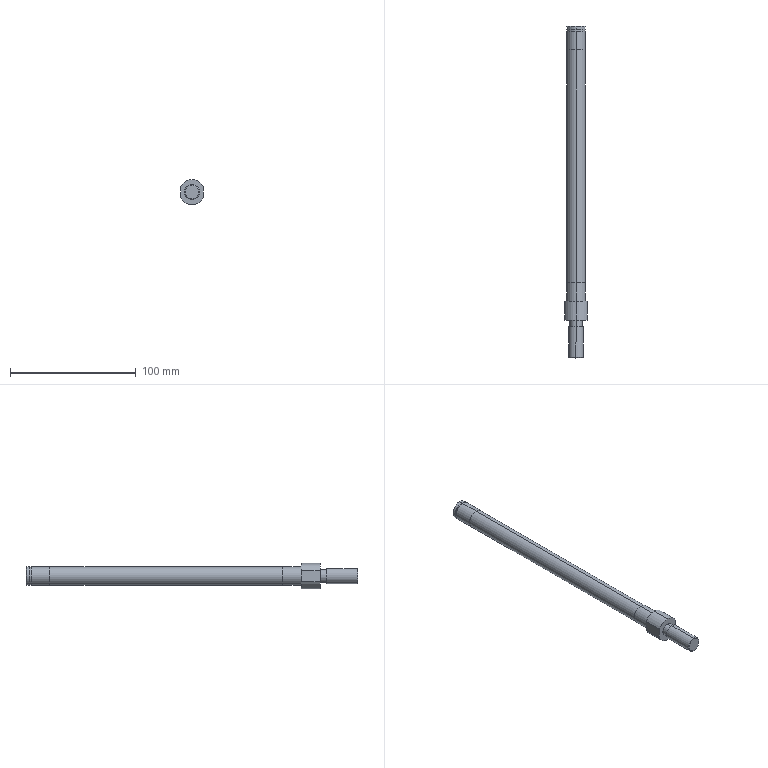Component | SolidWorks | 8TC-A15004-83-00-16_8TC-A15004-80-14A-1 | 1 solid | 32 faces | box 18 x 264 x 20 mm | volume 44695 mm3 | cylinder 17 | plane 11 | cone 4 | commonest cylinder face diameters 15 x6 20 x3 13.8 x2 14.6 x2 10 x2 12 x2 | material #45
build123d program:
from build123d import *

# Parameters (mm, degrees)
SKETCH2_OUTSIDE_W   = 75.102
SKETCH2_OUTSIDE_H   = 75.102
SKETCH2_OUTSIDE_W_2 = 24
SKETCH2_OUTSIDE_H_2 = 18
CUT_EXTRUDE1_DEPTH  = 264


with BuildPart() as part:
    # Sketch1 → Revolve1 (revolve)
    with BuildSketch(Plane(origin=(0, 0, 0), x_dir=(1, 0, 0), z_dir=(0, 1, 0)), mode=Mode.PRIVATE) as revolve1_sk:
        Polygon((0, 0), (0, 5.5), (0.5, 6), (25, 6), (25, 5), (30, 5), (30, 10), (45, 10), (45, 7.5), (60, 7.5), (60, 7.3), (245, 7.3), (245, 7.5), (260, 7.5), (260, 6.9), (261.15, 6.9), (261.15, 7.5), (263.5, 7.5), (264, 7), (264, 0), align=None)
    revolve(revolve1_sk.sketch.rotate(Axis((0, 0, 0), (1, 0, 0)), 180), axis=Axis((0, 0, 0), (1, 0, 0)))

    # Sketch2 outside → Cut-Extrude1 (cut)
    with BuildSketch(Plane.ZY):
        Rectangle(SKETCH2_OUTSIDE_W, SKETCH2_OUTSIDE_H)
        Rectangle(SKETCH2_OUTSIDE_W_2, SKETCH2_OUTSIDE_H_2, mode=Mode.SUBTRACT)
    extrude(amount=-CUT_EXTRUDE1_DEPTH, mode=Mode.SUBTRACT)


solid = part.part

# Placed as in the assembly
solid = solid.moved(Location((40, -22.5, 60), (0, 0, 90)))
STEP:
#1=COLOUR_RGB('',0.7922,0.8196,0.9333);
#2=FILL_AREA_STYLE_COLOUR('',#1);
#3=FILL_AREA_STYLE('',(#2));
#4=SURFACE_STYLE_FILL_AREA(#3);
#5=SURFACE_SIDE_STYLE('',(#4));
#6=SURFACE_STYLE_USAGE(.BOTH.,#5);
#7=PRESENTATION_STYLE_ASSIGNMENT((#6));
#8=CARTESIAN_POINT('',(1.575,9.508,2.638));
#9=VERTEX_POINT('',#8);
#10=CARTESIAN_POINT('',(1.575,9.508,2.087));
#11=VERTEX_POINT('',#10);
#12=CARTESIAN_POINT('',(1.575,9.508,2.362));
#13=DIRECTION('',(-0.,-1.,0.));
#14=DIRECTION('',(0.,0.,1.));
#15=AXIS2_PLACEMENT_3D('',#12,#13,#14);
#16=CIRCLE('',#15,0.2756);
#17=EDGE_CURVE('',#9,#11,#16,.T.);
#18=ORIENTED_EDGE('',*,*,#17,.T.);
#19=CARTESIAN_POINT('',(1.575,9.488,2.067));
#20=VERTEX_POINT('',#19);
#21=CARTESIAN_POINT('',(1.575,9.508,2.087));
#22=DIRECTION('',(-0.,-0.7071,-0.7071));
#23=VECTOR('',#22,39.37);
#24=LINE('',#21,#23);
#25=EDGE_CURVE('',#11,#20,#24,.T.);
#26=ORIENTED_EDGE('',*,*,#25,.T.);
#27=CARTESIAN_POINT('',(1.575,9.488,2.657));
#28=VERTEX_POINT('',#27);
#29=CARTESIAN_POINT('',(1.575,9.488,2.362));
#30=DIRECTION('',(-0.,-1.,0.));
#31=DIRECTION('',(0.,0.,1.));
#32=AXIS2_PLACEMENT_3D('',#29,#30,#31);
#33=CIRCLE('',#32,0.2953);
#34=EDGE_CURVE('',#28,#20,#33,.T.);
#35=ORIENTED_EDGE('',*,*,#34,.F.);
#36=CARTESIAN_POINT('',(1.575,9.508,2.638));
#37=DIRECTION('',(-0.,-0.7071,0.7071));
#38=VECTOR('',#37,39.37);
#39=LINE('',#36,#38);
#40=EDGE_CURVE('',#9,#28,#39,.T.);
#41=ORIENTED_EDGE('',*,*,#40,.F.);
#42=EDGE_LOOP('',(#18,#26,#35,#41));
#43=FACE_OUTER_BOUND('',#42,.T.);
#44=CARTESIAN_POINT('',(1.575,9.508,2.362));
#45=DIRECTION('',(-0.,-1.,0.));
#46=DIRECTION('',(0.,0.,1.));
#47=AXIS2_PLACEMENT_3D('',#44,#45,#46);
#48=CONICAL_SURFACE('',#47,0.2756,0.7854);
#49=ADVANCED_FACE('',(#43),#48,.T.);
#50=ORIENTED_EDGE('',*,*,#34,.T.);
#51=CARTESIAN_POINT('',(1.575,9.396,2.067));
#52=VERTEX_POINT('',#51);
#53=CARTESIAN_POINT('',(1.575,-0.8858,2.067));
#54=DIRECTION('',(-0.,-1.,0.));
#55=VECTOR('',#54,39.37);
#56=LINE('',#53,#55);
#57=EDGE_CURVE('',#20,#52,#56,.T.);
#58=ORIENTED_EDGE('',*,*,#57,.T.);
#59=CARTESIAN_POINT('',(1.575,9.396,2.657));
#60=VERTEX_POINT('',#59);
#61=CARTESIAN_POINT('',(1.575,9.396,2.362));
#62=DIRECTION('',(-0.,-1.,0.));
#63=DIRECTION('',(0.,0.,1.));
#64=AXIS2_PLACEMENT_3D('',#61,#62,#63);
#65=CIRCLE('',#64,0.2953);
#66=EDGE_CURVE('',#60,#52,#65,.T.);
#67=ORIENTED_EDGE('',*,*,#66,.F.);
#68=CARTESIAN_POINT('',(1.575,-0.8858,2.657));
#69=DIRECTION('',(-0.,-1.,0.));
#70=VECTOR('',#69,39.37);
#71=LINE('',#68,#70);
#72=EDGE_CURVE('',#28,#60,#71,.T.);
#73=ORIENTED_EDGE('',*,*,#72,.F.);
#74=EDGE_LOOP('',(#50,#58,#67,#73));
#75=FACE_OUTER_BOUND('',#74,.T.);
#76=CARTESIAN_POINT('',(1.575,-0.8858,2.362));
#77=DIRECTION('',(-0.,-1.,0.));
#78=DIRECTION('',(0.,0.,1.));
#79=AXIS2_PLACEMENT_3D('',#76,#77,#78);
#80=CYLINDRICAL_SURFACE('',#79,0.2953);
#81=ADVANCED_FACE('',(#75),#80,.T.);
#82=CARTESIAN_POINT('',(1.575,9.396,2.634));
#83=VERTEX_POINT('',#82);
#84=CARTESIAN_POINT('',(1.575,9.396,2.091));
#85=VERTEX_POINT('',#84);
#86=CARTESIAN_POINT('',(1.575,9.396,2.362));
#87=DIRECTION('',(-0.,-1.,0.));
#88=DIRECTION('',(0.,0.,1.));
#89=AXIS2_PLACEMENT_3D('',#86,#87,#88);
#90=CIRCLE('',#89,0.2717);
#91=EDGE_CURVE('',#83,#85,#90,.T.);
#92=ORIENTED_EDGE('',*,*,#91,.T.);
#93=CARTESIAN_POINT('',(1.575,9.35,2.091));
#94=VERTEX_POINT('',#93);
#95=CARTESIAN_POINT('',(1.575,-0.8858,2.091));
#96=DIRECTION('',(-0.,-1.,0.));
#97=VECTOR('',#96,39.37);
#98=LINE('',#95,#97);
#99=EDGE_CURVE('',#85,#94,#98,.T.);
#100=ORIENTED_EDGE('',*,*,#99,.T.);
#101=CARTESIAN_POINT('',(1.575,9.35,2.634));
#102=VERTEX_POINT('',#101);
#103=CARTESIAN_POINT('',(1.575,9.35,2.362));
#104=DIRECTION('',(-0.,-1.,0.));
#105=DIRECTION('',(0.,0.,1.));
#106=AXIS2_PLACEMENT_3D('',#103,#104,#105);
#107=CIRCLE('',#106,0.2717);
#108=EDGE_CURVE('',#102,#94,#107,.T.);
#109=ORIENTED_EDGE('',*,*,#108,.F.);
#110=CARTESIAN_POINT('',(1.575,-0.8858,2.634));
#111=DIRECTION('',(-0.,-1.,0.));
#112=VECTOR('',#111,39.37);
#113=LINE('',#110,#112);
#114=EDGE_CURVE('',#83,#102,#113,.T.);
#115=ORIENTED_EDGE('',*,*,#114,.F.);
#116=EDGE_LOOP('',(#92,#100,#109,#115));
#117=FACE_OUTER_BOUND('',#116,.T.);
#118=CARTESIAN_POINT('',(1.575,-0.8858,2.362));
#119=DIRECTION('',(-0.,-1.,0.));
#120=DIRECTION('',(0.,0.,1.));
#121=AXIS2_PLACEMENT_3D('',#118,#119,#120);
#122=CYLINDRICAL_SURFACE('',#121,0.2717);
#123=ADVANCED_FACE('',(#117),#122,.T.);
#124=CARTESIAN_POINT('',(1.575,9.35,2.657));
#125=VERTEX_POINT('',#124);
#126=CARTESIAN_POINT('',(1.575,9.35,2.067));
#127=VERTEX_POINT('',#126);
#128=CARTESIAN_POINT('',(1.575,9.35,2.362));
#129=DIRECTION('',(-0.,-1.,0.));
#130=DIRECTION('',(0.,0.,1.));
#131=AXIS2_PLACEMENT_3D('',#128,#129,#130);
#132=CIRCLE('',#131,0.2953);
#133=EDGE_CURVE('',#125,#127,#132,.T.);
#134=ORIENTED_EDGE('',*,*,#133,.T.);
#135=CARTESIAN_POINT('',(1.575,8.76,2.067));
#136=VERTEX_POINT('',#135);
#137=CARTESIAN_POINT('',(1.575,-0.8858,2.067));
#138=DIRECTION('',(-0.,-1.,0.));
#139=VECTOR('',#138,39.37);
#140=LINE('',#137,#139);
#141=EDGE_CURVE('',#127,#136,#140,.T.);
#142=ORIENTED_EDGE('',*,*,#141,.T.);
#143=CARTESIAN_POINT('',(1.575,8.76,2.657));
#144=VERTEX_POINT('',#143);
#145=CARTESIAN_POINT('',(1.575,8.76,2.362));
#146=DIRECTION('',(-0.,-1.,0.));
#147=DIRECTION('',(0.,0.,1.));
#148=AXIS2_PLACEMENT_3D('',#145,#146,#147);
#149=CIRCLE('',#148,0.2953);
#150=EDGE_CURVE('',#144,#136,#149,.T.);
#151=ORIENTED_EDGE('',*,*,#150,.F.);
#152=CARTESIAN_POINT('',(1.575,-0.8858,2.657));
#153=DIRECTION('',(-0.,-1.,0.));
#154=VECTOR('',#153,39.37);
#155=LINE('',#152,#154);
#156=EDGE_CURVE('',#125,#144,#155,.T.);
#157=ORIENTED_EDGE('',*,*,#156,.F.);
#158=EDGE_LOOP('',(#134,#142,#151,#157));
#159=FACE_OUTER_BOUND('',#158,.T.);
#160=CARTESIAN_POINT('',(1.575,-0.8858,2.362));
#161=DIRECTION('',(-0.,-1.,0.));
#162=DIRECTION('',(0.,0.,1.));
#163=AXIS2_PLACEMENT_3D('',#160,#161,#162);
#164=CYLINDRICAL_SURFACE('',#163,0.2953);
#165=ADVANCED_FACE('',(#159),#164,.T.);
#166=CARTESIAN_POINT('',(1.575,8.76,2.65));
#167=VERTEX_POINT('',#166);
#168=CARTESIAN_POINT('',(1.575,8.76,2.075));
#169=VERTEX_POINT('',#168);
#170=CARTESIAN_POINT('',(1.575,8.76,2.362));
#171=DIRECTION('',(-0.,-1.,0.));
#172=DIRECTION('',(0.,0.,1.));
#173=AXIS2_PLACEMENT_3D('',#170,#171,#172);
#174=CIRCLE('',#173,0.2874);
#175=EDGE_CURVE('',#167,#169,#174,.T.);
#176=ORIENTED_EDGE('',*,*,#175,.T.);
#177=CARTESIAN_POINT('',(1.575,1.476,2.075));
#178=VERTEX_POINT('',#177);
#179=CARTESIAN_POINT('',(1.575,-0.8858,2.075));
#180=DIRECTION('',(-0.,-1.,0.));
#181=VECTOR('',#180,39.37);
#182=LINE('',#179,#181);
#183=EDGE_CURVE('',#169,#178,#182,.T.);
#184=ORIENTED_EDGE('',*,*,#183,.T.);
#185=CARTESIAN_POINT('',(1.575,1.476,2.65));
#186=VERTEX_POINT('',#185);
#187=CARTESIAN_POINT('',(1.575,1.476,2.362));
#188=DIRECTION('',(-0.,-1.,0.));
#189=DIRECTION('',(0.,0.,1.));
#190=AXIS2_PLACEMENT_3D('',#187,#188,#189);
#191=CIRCLE('',#190,0.2874);
#192=EDGE_CURVE('',#186,#178,#191,.T.);
#193=ORIENTED_EDGE('',*,*,#192,.F.);
#194=CARTESIAN_POINT('',(1.575,-0.8858,2.65));
#195=DIRECTION('',(-0.,-1.,0.));
#196=VECTOR('',#195,39.37);
#197=LINE('',#194,#196);
#198=EDGE_CURVE('',#167,#186,#197,.T.);
#199=ORIENTED_EDGE('',*,*,#198,.F.);
#200=EDGE_LOOP('',(#176,#184,#193,#199));
#201=FACE_OUTER_BOUND('',#200,.T.);
#202=CARTESIAN_POINT('',(1.575,-0.8858,2.362));
#203=DIRECTION('',(-0.,-1.,0.));
#204=DIRECTION('',(0.,0.,1.));
#205=AXIS2_PLACEMENT_3D('',#202,#203,#204);
#206=CYLINDRICAL_SURFACE('',#205,0.2874);
#207=ADVANCED_FACE('',(#201),#206,.T.);
#208=CARTESIAN_POINT('',(1.575,1.476,2.657));
#209=VERTEX_POINT('',#208);
#210=CARTESIAN_POINT('',(1.575,1.476,2.067));
#211=VERTEX_POINT('',#210);
#212=CARTESIAN_POINT('',(1.575,1.476,2.362));
#213=DIRECTION('',(-0.,-1.,0.));
#214=DIRECTION('',(0.,0.,1.));
#215=AXIS2_PLACEMENT_3D('',#212,#213,#214);
#216=CIRCLE('',#215,0.2953);
#217=EDGE_CURVE('',#209,#211,#216,.T.);
#218=ORIENTED_EDGE('',*,*,#217,.T.);
#219=CARTESIAN_POINT('',(1.575,0.8858,2.067));
#220=VERTEX_POINT('',#219);
#221=CARTESIAN_POINT('',(1.575,-0.8858,2.067));
#222=DIRECTION('',(-0.,-1.,0.));
#223=VECTOR('',#222,39.37);
#224=LINE('',#221,#223);
#225=EDGE_CURVE('',#211,#220,#224,.T.);
#226=ORIENTED_EDGE('',*,*,#225,.T.);
#227=CARTESIAN_POINT('',(1.575,0.8858,2.657));
#228=VERTEX_POINT('',#227);
#229=CARTESIAN_POINT('',(1.575,0.8858,2.362));
#230=DIRECTION('',(-0.,-1.,0.));
#231=DIRECTION('',(0.,0.,1.));
#232=AXIS2_PLACEMENT_3D('',#229,#230,#231);
#233=CIRCLE('',#232,0.2953);
#234=EDGE_CURVE('',#228,#220,#233,.T.);
#235=ORIENTED_EDGE('',*,*,#234,.F.);
#236=CARTESIAN_POINT('',(1.575,-0.8858,2.657));
#237=DIRECTION('',(-0.,-1.,0.));
#238=VECTOR('',#237,39.37);
#239=LINE('',#236,#238);
#240=EDGE_CURVE('',#209,#228,#239,.T.);
#241=ORIENTED_EDGE('',*,*,#240,.F.);
#242=EDGE_LOOP('',(#218,#226,#235,#241));
#243=FACE_OUTER_BOUND('',#242,.T.);
#244=CARTESIAN_POINT('',(1.575,-0.8858,2.362));
#245=DIRECTION('',(-0.,-1.,0.));
#246=DIRECTION('',(0.,0.,1.));
#247=AXIS2_PLACEMENT_3D('',#244,#245,#246);
#248=CYLINDRICAL_SURFACE('',#247,0.2953);
#249=ADVANCED_FACE('',(#243),#248,.T.);
#250=CARTESIAN_POINT('',(1.929,0.8858,2.534));
#251=VERTEX_POINT('',#250);
#252=CARTESIAN_POINT('',(1.575,0.8858,2.756));
#253=VERTEX_POINT('',#252);
#254=CARTESIAN_POINT('',(1.575,0.8858,2.362));
#255=DIRECTION('',(-0.,-1.,0.));
#256=DIRECTION('',(0.,0.,1.));
#257=AXIS2_PLACEMENT_3D('',#254,#255,#256);
#258=CIRCLE('',#257,0.3937);
#259=EDGE_CURVE('',#251,#253,#258,.T.);
#260=ORIENTED_EDGE('',*,*,#259,.T.);
#261=CARTESIAN_POINT('',(1.575,0.2953,2.756));
#262=VERTEX_POINT('',#261);
#263=CARTESIAN_POINT('',(1.575,-0.8858,2.756));
#264=DIRECTION('',(-0.,-1.,0.));
#265=VECTOR('',#264,39.37);
#266=LINE('',#263,#265);
#267=EDGE_CURVE('',#253,#262,#266,.T.);
#268=ORIENTED_EDGE('',*,*,#267,.T.);
#269=CARTESIAN_POINT('',(1.929,0.2953,2.534));
#270=VERTEX_POINT('',#269);
#271=CARTESIAN_POINT('',(1.575,0.2953,2.362));
#272=DIRECTION('',(-0.,-1.,0.));
#273=DIRECTION('',(0.,0.,1.));
#274=AXIS2_PLACEMENT_3D('',#271,#272,#273);
#275=CIRCLE('',#274,0.3937);
#276=EDGE_CURVE('',#270,#262,#275,.T.);
#277=ORIENTED_EDGE('',*,*,#276,.F.);
#278=CARTESIAN_POINT('',(1.929,-0.8858,2.534));
#279=DIRECTION('',(0.,1.,0.));
#280=VECTOR('',#279,39.37);
#281=LINE('',#278,#280);
#282=EDGE_CURVE('',#270,#251,#281,.T.);
#283=ORIENTED_EDGE('',*,*,#282,.T.);
#284=EDGE_LOOP('',(#260,#268,#277,#283));
#285=FACE_OUTER_BOUND('',#284,.T.);
#286=CARTESIAN_POINT('',(1.575,-0.8858,2.362));
#287=DIRECTION('',(-0.,-1.,0.));
#288=DIRECTION('',(0.,0.,1.));
#289=AXIS2_PLACEMENT_3D('',#286,#287,#288);
#290=CYLINDRICAL_SURFACE('',#289,0.3937);
#291=ADVANCED_FACE('',(#285),#290,.T.);
#292=CARTESIAN_POINT('',(1.575,0.2953,2.559));
#293=VERTEX_POINT('',#292);
#294=CARTESIAN_POINT('',(1.575,0.2953,2.165));
#295=VERTEX_POINT('',#294);
#296=CARTESIAN_POINT('',(1.575,0.2953,2.362));
#297=DIRECTION('',(-0.,-1.,0.));
#298=DIRECTION('',(0.,0.,1.));
#299=AXIS2_PLACEMENT_3D('',#296,#297,#298);
#300=CIRCLE('',#299,0.1969);
#301=EDGE_CURVE('',#293,#295,#300,.T.);
#302=ORIENTED_EDGE('',*,*,#301,.T.);
#303=CARTESIAN_POINT('',(1.575,0.09843,2.165));
#304=VERTEX_POINT('',#303);
#305=CARTESIAN_POINT('',(1.575,-0.8858,2.165));
#306=DIRECTION('',(-0.,-1.,0.));
#307=VECTOR('',#306,39.37);
#308=LINE('',#305,#307);
#309=EDGE_CURVE('',#295,#304,#308,.T.);
#310=ORIENTED_EDGE('',*,*,#309,.T.);
#311=CARTESIAN_POINT('',(1.575,0.09843,2.559));
#312=VERTEX_POINT('',#311);
#313=CARTESIAN_POINT('',(1.575,0.09843,2.362));
#314=DIRECTION('',(-0.,-1.,0.));
#315=DIRECTION('',(0.,0.,1.));
#316=AXIS2_PLACEMENT_3D('',#313,#314,#315);
#317=CIRCLE('',#316,0.1969);
#318=EDGE_CURVE('',#312,#304,#317,.T.);
#319=ORIENTED_EDGE('',*,*,#318,.F.);
#320=CARTESIAN_POINT('',(1.575,-0.8858,2.559));
#321=DIRECTION('',(-0.,-1.,0.));
#322=VECTOR('',#321,39.37);
#323=LINE('',#320,#322);
#324=EDGE_CURVE('',#293,#312,#323,.T.);
#325=ORIENTED_EDGE('',*,*,#324,.F.);
#326=EDGE_LOOP('',(#302,#310,#319,#325));
#327=FACE_OUTER_BOUND('',#326,.T.);
#328=CARTESIAN_POINT('',(1.575,-0.8858,2.362));
#329=DIRECTION('',(-0.,-1.,0.));
#330=DIRECTION('',(0.,0.,1.));
#331=AXIS2_PLACEMENT_3D('',#328,#329,#330);
#332=CYLINDRICAL_SURFACE('',#331,0.1969);
#333=ADVANCED_FACE('',(#327),#332,.T.);
#334=CARTESIAN_POINT('',(1.575,0.09843,2.598));
#335=VERTEX_POINT('',#334);
#336=CARTESIAN_POINT('',(1.575,0.09843,2.126));
#337=VERTEX_POINT('',#336);
#338=CARTESIAN_POINT('',(1.575,0.09843,2.362));
#339=DIRECTION('',(-0.,-1.,0.));
#340=DIRECTION('',(0.,0.,1.));
#341=AXIS2_PLACEMENT_3D('',#338,#339,#340);
#342=CIRCLE('',#341,0.2362);
#343=EDGE_CURVE('',#335,#337,#342,.T.);
#344=ORIENTED_EDGE('',*,*,#343,.T.);
#345=CARTESIAN_POINT('',(1.575,-0.8661,2.126));
#346=VERTEX_POINT('',#345);
#347=CARTESIAN_POINT('',(1.575,-0.8858,2.126));
#348=DIRECTION('',(-0.,-1.,0.));
#349=VECTOR('',#348,39.37);
#350=LINE('',#347,#349);
#351=EDGE_CURVE('',#337,#346,#350,.T.);
#352=ORIENTED_EDGE('',*,*,#351,.T.);
#353=CARTESIAN_POINT('',(1.575,-0.8661,2.598));
#354=VERTEX_POINT('',#353);
#355=CARTESIAN_POINT('',(1.575,-0.8661,2.362));
#356=DIRECTION('',(-0.,-1.,0.));
#357=DIRECTION('',(0.,0.,1.));
#358=AXIS2_PLACEMENT_3D('',#355,#356,#357);
#359=CIRCLE('',#358,0.2362);
#360=EDGE_CURVE('',#354,#346,#359,.T.);
#361=ORIENTED_EDGE('',*,*,#360,.F.);
#362=CARTESIAN_POINT('',(1.575,-0.8858,2.598));
#363=DIRECTION('',(-0.,-1.,0.));
#364=VECTOR('',#363,39.37);
#365=LINE('',#362,#364);
#366=EDGE_CURVE('',#335,#354,#365,.T.);
#367=ORIENTED_EDGE('',*,*,#366,.F.);
#368=EDGE_LOOP('',(#344,#352,#361,#367));
#369=FACE_OUTER_BOUND('',#368,.T.);
#370=CARTESIAN_POINT('',(1.575,-0.8858,2.362));
#371=DIRECTION('',(-0.,-1.,0.));
#372=DIRECTION('',(0.,0.,1.));
#373=AXIS2_PLACEMENT_3D('',#370,#371,#372);
#374=CYLINDRICAL_SURFACE('',#373,0.2362);
#375=ADVANCED_FACE('',(#369),#374,.T.);
#376=CARTESIAN_POINT('',(1.575,-0.8858,2.579));
#377=VERTEX_POINT('',#376);
#378=CARTESIAN_POINT('',(1.575,-0.8858,2.146));
#379=VERTEX_POINT('',#378);
#380=CARTESIAN_POINT('',(1.575,-0.8858,2.362));
#381=DIRECTION('',(-0.,-1.,0.));
#382=DIRECTION('',(0.,0.,1.));
#383=AXIS2_PLACEMENT_3D('',#380,#381,#382);
#384=CIRCLE('',#383,0.2165);
#385=EDGE_CURVE('',#377,#379,#384,.T.);
#386=ORIENTED_EDGE('',*,*,#385,.F.);
#387=CARTESIAN_POINT('',(1.575,-0.8661,2.598));
#388=DIRECTION('',(0.,0.7071,0.7071));
#389=VECTOR('',#388,39.37);
#390=LINE('',#387,#389);
#391=EDGE_CURVE('',#377,#354,#390,.T.);
#392=ORIENTED_EDGE('',*,*,#391,.T.);
#393=ORIENTED_EDGE('',*,*,#360,.T.);
#394=CARTESIAN_POINT('',(1.575,-0.8661,2.126));
#395=DIRECTION('',(0.,0.7071,-0.7071));
#396=VECTOR('',#395,39.37);
#397=LINE('',#394,#396);
#398=EDGE_CURVE('',#379,#346,#397,.T.);
#399=ORIENTED_EDGE('',*,*,#398,.F.);
#400=EDGE_LOOP('',(#386,#392,#393,#399));
#401=FACE_OUTER_BOUND('',#400,.T.);
#402=CARTESIAN_POINT('',(1.575,-0.8661,2.362));
#403=DIRECTION('',(0.,1.,0.));
#404=DIRECTION('',(0.,0.,-1.));
#405=AXIS2_PLACEMENT_3D('',#402,#403,#404);
#406=CONICAL_SURFACE('',#405,0.2362,0.7854);
#407=ADVANCED_FACE('',(#401),#406,.T.);
#408=CARTESIAN_POINT('',(1.22,0.2953,2.191));
#409=VERTEX_POINT('',#408);
#410=CARTESIAN_POINT('',(1.22,0.8858,2.191));
#411=VERTEX_POINT('',#410);
#412=CARTESIAN_POINT('',(1.22,-0.8858,2.191));
#413=DIRECTION('',(0.,1.,0.));
#414=VECTOR('',#413,39.37);
#415=LINE('',#412,#414);
#416=EDGE_CURVE('',#409,#411,#415,.T.);
#417=ORIENTED_EDGE('',*,*,#416,.T.);
#418=CARTESIAN_POINT('',(1.929,0.8858,2.191));
#419=VERTEX_POINT('',#418);
#420=CARTESIAN_POINT('',(1.575,0.8858,2.362));
#421=DIRECTION('',(-0.,-1.,0.));
#422=DIRECTION('',(0.,0.,1.));
#423=AXIS2_PLACEMENT_3D('',#420,#421,#422);
#424=CIRCLE('',#423,0.3937);
#425=EDGE_CURVE('',#411,#419,#424,.T.);
#426=ORIENTED_EDGE('',*,*,#425,.T.);
#427=CARTESIAN_POINT('',(1.929,0.2953,2.191));
#428=VERTEX_POINT('',#427);
#429=CARTESIAN_POINT('',(1.929,-0.8858,2.191));
#430=DIRECTION('',(-0.,-1.,0.));
#431=VECTOR('',#430,39.37);
#432=LINE('',#429,#431);
#433=EDGE_CURVE('',#419,#428,#432,.T.);
#434=ORIENTED_EDGE('',*,*,#433,.T.);
#435=CARTESIAN_POINT('',(1.575,0.2953,2.362));
#436=DIRECTION('',(-0.,-1.,0.));
#437=DIRECTION('',(0.,0.,1.));
#438=AXIS2_PLACEMENT_3D('',#435,#436,#437);
#439=CIRCLE('',#438,0.3937);
#440=EDGE_CURVE('',#409,#428,#439,.T.);
#441=ORIENTED_EDGE('',*,*,#440,.F.);
#442=EDGE_LOOP('',(#417,#426,#434,#441));
#443=FACE_OUTER_BOUND('',#442,.T.);
#444=CARTESIAN_POINT('',(1.575,-0.8858,2.362));
#445=DIRECTION('',(-0.,-1.,0.));
#446=DIRECTION('',(0.,0.,1.));
#447=AXIS2_PLACEMENT_3D('',#444,#445,#446);
#448=CYLINDRICAL_SURFACE('',#447,0.3937);
#449=ADVANCED_FACE('',(#443),#448,.T.);
#450=CARTESIAN_POINT('',(1.575,-0.8858,2.362));
#451=DIRECTION('',(-0.,-1.,0.));
#452=DIRECTION('',(0.,0.,1.));
#453=AXIS2_PLACEMENT_3D('',#450,#451,#452);
#454=CIRCLE('',#453,0.2165);
#455=EDGE_CURVE('',#379,#377,#454,.T.);
#456=ORIENTED_EDGE('',*,*,#455,.T.);
#457=ORIENTED_EDGE('',*,*,#385,.T.);
#458=EDGE_LOOP('',(#456,#457));
#459=FACE_OUTER_BOUND('',#458,.T.);
#460=CARTESIAN_POINT('',(1.575,-0.8858,2.362));
#461=DIRECTION('',(0.,1.,0.));
#462=DIRECTION('',(0.,0.,-1.));
#463=AXIS2_PLACEMENT_3D('',#460,#461,#462);
#464=PLANE('',#463);
#465=ADVANCED_FACE('',(#459),#464,.F.);
#466=ORIENTED_EDGE('',*,*,#391,.F.);
#467=ORIENTED_EDGE('',*,*,#455,.F.);
#468=ORIENTED_EDGE('',*,*,#398,.T.);
#469=CARTESIAN_POINT('',(1.575,-0.8661,2.362));
#470=DIRECTION('',(-0.,-1.,0.));
#471=DIRECTION('',(0.,0.,1.));
#472=AXIS2_PLACEMENT_3D('',#469,#470,#471);
#473=CIRCLE('',#472,0.2362);
#474=EDGE_CURVE('',#346,#354,#473,.T.);
#475=ORIENTED_EDGE('',*,*,#474,.T.);
#476=EDGE_LOOP('',(#466,#467,#468,#475));
#477=FACE_OUTER_BOUND('',#476,.T.);
#478=CARTESIAN_POINT('',(1.575,-0.8661,2.362));
#479=DIRECTION('',(0.,1.,0.));
#480=DIRECTION('',(0.,0.,-1.));
#481=AXIS2_PLACEMENT_3D('',#478,#479,#480);
#482=CONICAL_SURFACE('',#481,0.2362,0.7854);
#483=ADVANCED_FACE('',(#477),#482,.T.);
#484=ORIENTED_EDGE('',*,*,#351,.F.);
#485=CARTESIAN_POINT('',(1.575,0.09843,2.362));
#486=DIRECTION('',(-0.,-1.,0.));
#487=DIRECTION('',(0.,0.,1.));
#488=AXIS2_PLACEMENT_3D('',#485,#486,#487);
#489=CIRCLE('',#488,0.2362);
#490=EDGE_CURVE('',#337,#335,#489,.T.);
#491=ORIENTED_EDGE('',*,*,#490,.T.);
#492=ORIENTED_EDGE('',*,*,#366,.T.);
#493=ORIENTED_EDGE('',*,*,#474,.F.);
#494=EDGE_LOOP('',(#484,#491,#492,#493));
#495=FACE_OUTER_BOUND('',#494,.T.);
#496=CARTESIAN_POINT('',(1.575,-0.8858,2.362));
#497=DIRECTION('',(-0.,-1.,0.));
#498=DIRECTION('',(0.,0.,1.));
#499=AXIS2_PLACEMENT_3D('',#496,#497,#498);
#500=CYLINDRICAL_SURFACE('',#499,0.2362);
#501=ADVANCED_FACE('',(#495),#500,.T.);
#502=ORIENTED_EDGE('',*,*,#343,.F.);
#503=ORIENTED_EDGE('',*,*,#490,.F.);
#504=EDGE_LOOP('',(#502,#503));
#505=FACE_OUTER_BOUND('',#504,.T.);
#506=ORIENTED_EDGE('',*,*,#318,.T.);
#507=CARTESIAN_POINT('',(1.575,0.09843,2.362));
#508=DIRECTION('',(-0.,-1.,0.));
#509=DIRECTION('',(0.,0.,1.));
#510=AXIS2_PLACEMENT_3D('',#507,#508,#509);
#511=CIRCLE('',#510,0.1969);
#512=EDGE_CURVE('',#304,#312,#511,.T.);
#513=ORIENTED_EDGE('',*,*,#512,.T.);
#514=EDGE_LOOP('',(#506,#513));
#515=FACE_BOUND('',#514,.T.);
#516=CARTESIAN_POINT('',(1.575,0.09843,2.126));
#517=DIRECTION('',(-0.,-1.,0.));
#518=DIRECTION('',(0.,0.,1.));
#519=AXIS2_PLACEMENT_3D('',#516,#517,#518);
#520=PLANE('',#519);
#521=ADVANCED_FACE('',(#505,#515),#520,.F.);
#522=ORIENTED_EDGE('',*,*,#309,.F.);
#523=CARTESIAN_POINT('',(1.575,0.2953,2.362));
#524=DIRECTION('',(-0.,-1.,0.));
#525=DIRECTION('',(0.,0.,1.));
#526=AXIS2_PLACEMENT_3D('',#523,#524,#525);
#527=CIRCLE('',#526,0.1969);
#528=EDGE_CURVE('',#295,#293,#527,.T.);
#529=ORIENTED_EDGE('',*,*,#528,.T.);
#530=ORIENTED_EDGE('',*,*,#324,.T.);
#531=ORIENTED_EDGE('',*,*,#512,.F.);
#532=EDGE_LOOP('',(#522,#529,#530,#531));
#533=FACE_OUTER_BOUND('',#532,.T.);
#534=CARTESIAN_POINT('',(1.575,-0.8858,2.362));
#535=DIRECTION('',(-0.,-1.,0.));
#536=DIRECTION('',(0.,0.,1.));
#537=AXIS2_PLACEMENT_3D('',#534,#535,#536);
#538=CYLINDRICAL_SURFACE('',#537,0.1969);
#539=ADVANCED_FACE('',(#533),#538,.T.);
#540=CARTESIAN_POINT('',(1.22,0.2953,2.534));
#541=VERTEX_POINT('',#540);
#542=CARTESIAN_POINT('',(1.22,0.2953,1.89));
#543=DIRECTION('',(0.,0.,-1.));
#544=VECTOR('',#543,39.37);
#545=LINE('',#542,#544);
#546=EDGE_CURVE('',#541,#409,#545,.T.);
#547=ORIENTED_EDGE('',*,*,#546,.T.);
#548=ORIENTED_EDGE('',*,*,#440,.T.);
#549=CARTESIAN_POINT('',(1.929,0.2953,1.89));
#550=DIRECTION('',(0.,0.,1.));
#551=VECTOR('',#550,39.37);
#552=LINE('',#549,#551);
#553=EDGE_CURVE('',#428,#270,#552,.T.);
#554=ORIENTED_EDGE('',*,*,#553,.T.);
#555=ORIENTED_EDGE('',*,*,#276,.T.);
#556=CARTESIAN_POINT('',(1.575,0.2953,2.362));
#557=DIRECTION('',(-0.,-1.,0.));
#558=DIRECTION('',(0.,0.,1.));
#559=AXIS2_PLACEMENT_3D('',#556,#557,#558);
#560=CIRCLE('',#559,0.3937);
#561=EDGE_CURVE('',#262,#541,#560,.T.);
#562=ORIENTED_EDGE('',*,*,#561,.T.);
#563=EDGE_LOOP('',(#547,#548,#554,#555,#562));
#564=FACE_OUTER_BOUND('',#563,.T.);
#565=ORIENTED_EDGE('',*,*,#301,.F.);
#566=ORIENTED_EDGE('',*,*,#528,.F.);
#567=EDGE_LOOP('',(#565,#566));
#568=FACE_BOUND('',#567,.T.);
#569=CARTESIAN_POINT('',(1.575,0.2953,2.165));
#570=DIRECTION('',(0.,1.,0.));
#571=DIRECTION('',(0.,0.,-1.));
#572=AXIS2_PLACEMENT_3D('',#569,#570,#571);
#573=PLANE('',#572);
#574=ADVANCED_FACE('',(#564,#568),#573,.F.);
#575=ORIENTED_EDGE('',*,*,#267,.F.);
#576=CARTESIAN_POINT('',(1.22,0.8858,2.534));
#577=VERTEX_POINT('',#576);
#578=CARTESIAN_POINT('',(1.575,0.8858,2.362));
#579=DIRECTION('',(-0.,-1.,0.));
#580=DIRECTION('',(0.,0.,1.));
#581=AXIS2_PLACEMENT_3D('',#578,#579,#580);
#582=CIRCLE('',#581,0.3937);
#583=EDGE_CURVE('',#253,#577,#582,.T.);
#584=ORIENTED_EDGE('',*,*,#583,.T.);
#585=CARTESIAN_POINT('',(1.22,-0.8858,2.534));
#586=DIRECTION('',(-0.,-1.,0.));
#587=VECTOR('',#586,39.37);
#588=LINE('',#585,#587);
#589=EDGE_CURVE('',#577,#541,#588,.T.);
#590=ORIENTED_EDGE('',*,*,#589,.T.);
#591=ORIENTED_EDGE('',*,*,#561,.F.);
#592=EDGE_LOOP('',(#575,#584,#590,#591));
#593=FACE_OUTER_BOUND('',#592,.T.);
#594=CARTESIAN_POINT('',(1.575,-0.8858,2.362));
#595=DIRECTION('',(-0.,-1.,0.));
#596=DIRECTION('',(0.,0.,1.));
#597=AXIS2_PLACEMENT_3D('',#594,#595,#596);
#598=CYLINDRICAL_SURFACE('',#597,0.3937);
#599=ADVANCED_FACE('',(#593),#598,.T.);
#600=CARTESIAN_POINT('',(1.22,0.8858,1.89));
#601=DIRECTION('',(0.,0.,1.));
#602=VECTOR('',#601,39.37);
#603=LINE('',#600,#602);
#604=EDGE_CURVE('',#411,#577,#603,.T.);
#605=ORIENTED_EDGE('',*,*,#604,.T.);
#606=ORIENTED_EDGE('',*,*,#583,.F.);
#607=ORIENTED_EDGE('',*,*,#259,.F.);
#608=CARTESIAN_POINT('',(1.929,0.8858,1.89));
#609=DIRECTION('',(0.,0.,-1.));
#610=VECTOR('',#609,39.37);
#611=LINE('',#608,#610);
#612=EDGE_CURVE('',#251,#419,#611,.T.);
#613=ORIENTED_EDGE('',*,*,#612,.T.);
#614=ORIENTED_EDGE('',*,*,#425,.F.);
#615=EDGE_LOOP('',(#605,#606,#607,#613,#614));
#616=FACE_OUTER_BOUND('',#615,.T.);
#617=ORIENTED_EDGE('',*,*,#234,.T.);
#618=CARTESIAN_POINT('',(1.575,0.8858,2.362));
#619=DIRECTION('',(-0.,-1.,0.));
#620=DIRECTION('',(0.,0.,1.));
#621=AXIS2_PLACEMENT_3D('',#618,#619,#620);
#622=CIRCLE('',#621,0.2953);
#623=EDGE_CURVE('',#220,#228,#622,.T.);
#624=ORIENTED_EDGE('',*,*,#623,.T.);
#625=EDGE_LOOP('',(#617,#624));
#626=FACE_BOUND('',#625,.T.);
#627=CARTESIAN_POINT('',(1.575,0.8858,1.969));
#628=DIRECTION('',(-0.,-1.,0.));
#629=DIRECTION('',(0.,0.,1.));
#630=AXIS2_PLACEMENT_3D('',#627,#628,#629);
#631=PLANE('',#630);
#632=ADVANCED_FACE('',(#616,#626),#631,.F.);
#633=ORIENTED_EDGE('',*,*,#225,.F.);
#634=CARTESIAN_POINT('',(1.575,1.476,2.362));
#635=DIRECTION('',(-0.,-1.,0.));
#636=DIRECTION('',(0.,0.,1.));
#637=AXIS2_PLACEMENT_3D('',#634,#635,#636);
#638=CIRCLE('',#637,0.2953);
#639=EDGE_CURVE('',#211,#209,#638,.T.);
#640=ORIENTED_EDGE('',*,*,#639,.T.);
#641=ORIENTED_EDGE('',*,*,#240,.T.);
#642=ORIENTED_EDGE('',*,*,#623,.F.);
#643=EDGE_LOOP('',(#633,#640,#641,#642));
#644=FACE_OUTER_BOUND('',#643,.T.);
#645=CARTESIAN_POINT('',(1.575,-0.8858,2.362));
#646=DIRECTION('',(-0.,-1.,0.));
#647=DIRECTION('',(0.,0.,1.));
#648=AXIS2_PLACEMENT_3D('',#645,#646,#647);
#649=CYLINDRICAL_SURFACE('',#648,0.2953);
#650=ADVANCED_FACE('',(#644),#649,.T.);
#651=ORIENTED_EDGE('',*,*,#217,.F.);
#652=ORIENTED_EDGE('',*,*,#639,.F.);
#653=EDGE_LOOP('',(#651,#652));
#654=FACE_OUTER_BOUND('',#653,.T.);
#655=ORIENTED_EDGE('',*,*,#192,.T.);
#656=CARTESIAN_POINT('',(1.575,1.476,2.362));
#657=DIRECTION('',(-0.,-1.,0.));
#658=DIRECTION('',(0.,0.,1.));
#659=AXIS2_PLACEMENT_3D('',#656,#657,#658);
#660=CIRCLE('',#659,0.2874);
#661=EDGE_CURVE('',#178,#186,#660,.T.);
#662=ORIENTED_EDGE('',*,*,#661,.T.);
#663=EDGE_LOOP('',(#655,#662));
#664=FACE_BOUND('',#663,.T.);
#665=CARTESIAN_POINT('',(1.575,1.476,2.067));
#666=DIRECTION('',(-0.,-1.,0.));
#667=DIRECTION('',(0.,0.,1.));
#668=AXIS2_PLACEMENT_3D('',#665,#666,#667);
#669=PLANE('',#668);
#670=ADVANCED_FACE('',(#654,#664),#669,.F.);
#671=ORIENTED_EDGE('',*,*,#183,.F.);
#672=CARTESIAN_POINT('',(1.575,8.76,2.362));
#673=DIRECTION('',(-0.,-1.,0.));
#674=DIRECTION('',(0.,0.,1.));
#675=AXIS2_PLACEMENT_3D('',#672,#673,#674);
#676=CIRCLE('',#675,0.2874);
#677=EDGE_CURVE('',#169,#167,#676,.T.);
#678=ORIENTED_EDGE('',*,*,#677,.T.);
#679=ORIENTED_EDGE('',*,*,#198,.T.);
#680=ORIENTED_EDGE('',*,*,#661,.F.);
#681=EDGE_LOOP('',(#671,#678,#679,#680));
#682=FACE_OUTER_BOUND('',#681,.T.);
#683=CARTESIAN_POINT('',(1.575,-0.8858,2.362));
#684=DIRECTION('',(-0.,-1.,0.));
#685=DIRECTION('',(0.,0.,1.));
#686=AXIS2_PLACEMENT_3D('',#683,#684,#685);
#687=CYLINDRICAL_SURFACE('',#686,0.2874);
#688=ADVANCED_FACE('',(#682),#687,.T.);
#689=ORIENTED_EDGE('',*,*,#175,.F.);
#690=ORIENTED_EDGE('',*,*,#677,.F.);
#691=EDGE_LOOP('',(#689,#690));
#692=FACE_BOUND('',#691,.T.);
#693=ORIENTED_EDGE('',*,*,#150,.T.);
#694=CARTESIAN_POINT('',(1.575,8.76,2.362));
#695=DIRECTION('',(-0.,-1.,0.));
#696=DIRECTION('',(0.,0.,1.));
#697=AXIS2_PLACEMENT_3D('',#694,#695,#696);
#698=CIRCLE('',#697,0.2953);
#699=EDGE_CURVE('',#136,#144,#698,.T.);
#700=ORIENTED_EDGE('',*,*,#699,.T.);
#701=EDGE_LOOP('',(#693,#700));
#702=FACE_OUTER_BOUND('',#701,.T.);
#703=CARTESIAN_POINT('',(1.575,8.76,2.075));
#704=DIRECTION('',(0.,1.,0.));
#705=DIRECTION('',(0.,0.,-1.));
#706=AXIS2_PLACEMENT_3D('',#703,#704,#705);
#707=PLANE('',#706);
#708=ADVANCED_FACE('',(#692,#702),#707,.F.);
#709=ORIENTED_EDGE('',*,*,#141,.F.);
#710=CARTESIAN_POINT('',(1.575,9.35,2.362));
#711=DIRECTION('',(-0.,-1.,0.));
#712=DIRECTION('',(0.,0.,1.));
#713=AXIS2_PLACEMENT_3D('',#710,#711,#712);
#714=CIRCLE('',#713,0.2953);
#715=EDGE_CURVE('',#127,#125,#714,.T.);
#716=ORIENTED_EDGE('',*,*,#715,.T.);
#717=ORIENTED_EDGE('',*,*,#156,.T.);
#718=ORIENTED_EDGE('',*,*,#699,.F.);
#719=EDGE_LOOP('',(#709,#716,#717,#718));
#720=FACE_OUTER_BOUND('',#719,.T.);
#721=CARTESIAN_POINT('',(1.575,-0.8858,2.362));
#722=DIRECTION('',(-0.,-1.,0.));
#723=DIRECTION('',(0.,0.,1.));
#724=AXIS2_PLACEMENT_3D('',#721,#722,#723);
#725=CYLINDRICAL_SURFACE('',#724,0.2953);
#726=ADVANCED_FACE('',(#720),#725,.T.);
#727=ORIENTED_EDGE('',*,*,#133,.F.);
#728=ORIENTED_EDGE('',*,*,#715,.F.);
#729=EDGE_LOOP('',(#727,#728));
#730=FACE_OUTER_BOUND('',#729,.T.);
#731=ORIENTED_EDGE('',*,*,#108,.T.);
#732=CARTESIAN_POINT('',(1.575,9.35,2.362));
#733=DIRECTION('',(-0.,-1.,0.));
#734=DIRECTION('',(0.,0.,1.));
#735=AXIS2_PLACEMENT_3D('',#732,#733,#734);
#736=CIRCLE('',#735,0.2717);
#737=EDGE_CURVE('',#94,#102,#736,.T.);
#738=ORIENTED_EDGE('',*,*,#737,.T.);
#739=EDGE_LOOP('',(#731,#738));
#740=FACE_BOUND('',#739,.T.);
#741=CARTESIAN_POINT('',(1.575,9.35,2.067));
#742=DIRECTION('',(-0.,-1.,0.));
#743=DIRECTION('',(0.,0.,1.));
#744=AXIS2_PLACEMENT_3D('',#741,#742,#743);
#745=PLANE('',#744);
#746=ADVANCED_FACE('',(#730,#740),#745,.F.);
#747=ORIENTED_EDGE('',*,*,#99,.F.);
#748=CARTESIAN_POINT('',(1.575,9.396,2.362));
#749=DIRECTION('',(-0.,-1.,0.));
#750=DIRECTION('',(0.,0.,1.));
#751=AXIS2_PLACEMENT_3D('',#748,#749,#750);
#752=CIRCLE('',#751,0.2717);
#753=EDGE_CURVE('',#85,#83,#752,.T.);
#754=ORIENTED_EDGE('',*,*,#753,.T.);
#755=ORIENTED_EDGE('',*,*,#114,.T.);
#756=ORIENTED_EDGE('',*,*,#737,.F.);
#757=EDGE_LOOP('',(#747,#754,#755,#756));
#758=FACE_OUTER_BOUND('',#757,.T.);
#759=CARTESIAN_POINT('',(1.575,-0.8858,2.362));
#760=DIRECTION('',(-0.,-1.,0.));
#761=DIRECTION('',(0.,0.,1.));
#762=AXIS2_PLACEMENT_3D('',#759,#760,#761);
#763=CYLINDRICAL_SURFACE('',#762,0.2717);
#764=ADVANCED_FACE('',(#758),#763,.T.);
#765=ORIENTED_EDGE('',*,*,#91,.F.);
#766=ORIENTED_EDGE('',*,*,#753,.F.);
#767=EDGE_LOOP('',(#765,#766));
#768=FACE_BOUND('',#767,.T.);
#769=ORIENTED_EDGE('',*,*,#66,.T.);
#770=CARTESIAN_POINT('',(1.575,9.396,2.362));
#771=DIRECTION('',(-0.,-1.,0.));
#772=DIRECTION('',(0.,0.,1.));
#773=AXIS2_PLACEMENT_3D('',#770,#771,#772);
#774=CIRCLE('',#773,0.2953);
#775=EDGE_CURVE('',#52,#60,#774,.T.);
#776=ORIENTED_EDGE('',*,*,#775,.T.);
#777=EDGE_LOOP('',(#769,#776));
#778=FACE_OUTER_BOUND('',#777,.T.);
#779=CARTESIAN_POINT('',(1.575,9.396,2.091));
#780=DIRECTION('',(0.,1.,0.));
#781=DIRECTION('',(0.,0.,-1.));
#782=AXIS2_PLACEMENT_3D('',#779,#780,#781);
#783=PLANE('',#782);
#784=ADVANCED_FACE('',(#768,#778),#783,.F.);
#785=ORIENTED_EDGE('',*,*,#57,.F.);
#786=CARTESIAN_POINT('',(1.575,9.488,2.362));
#787=DIRECTION('',(-0.,-1.,0.));
#788=DIRECTION('',(0.,0.,1.));
#789=AXIS2_PLACEMENT_3D('',#786,#787,#788);
#790=CIRCLE('',#789,0.2953);
#791=EDGE_CURVE('',#20,#28,#790,.T.);
#792=ORIENTED_EDGE('',*,*,#791,.T.);
#793=ORIENTED_EDGE('',*,*,#72,.T.);
#794=ORIENTED_EDGE('',*,*,#775,.F.);
#795=EDGE_LOOP('',(#785,#792,#793,#794));
#796=FACE_OUTER_BOUND('',#795,.T.);
#797=CARTESIAN_POINT('',(1.575,-0.8858,2.362));
#798=DIRECTION('',(-0.,-1.,0.));
#799=DIRECTION('',(0.,0.,1.));
#800=AXIS2_PLACEMENT_3D('',#797,#798,#799);
#801=CYLINDRICAL_SURFACE('',#800,0.2953);
#802=ADVANCED_FACE('',(#796),#801,.T.);
#803=ORIENTED_EDGE('',*,*,#25,.F.);
#804=CARTESIAN_POINT('',(1.575,9.508,2.362));
#805=DIRECTION('',(-0.,-1.,0.));
#806=DIRECTION('',(0.,0.,1.));
#807=AXIS2_PLACEMENT_3D('',#804,#805,#806);
#808=CIRCLE('',#807,0.2756);
#809=EDGE_CURVE('',#11,#9,#808,.T.);
#810=ORIENTED_EDGE('',*,*,#809,.T.);
#811=ORIENTED_EDGE('',*,*,#40,.T.);
#812=ORIENTED_EDGE('',*,*,#791,.F.);
#813=EDGE_LOOP('',(#803,#810,#811,#812));
#814=FACE_OUTER_BOUND('',#813,.T.);
#815=CARTESIAN_POINT('',(1.575,9.508,2.362));
#816=DIRECTION('',(-0.,-1.,0.));
#817=DIRECTION('',(0.,0.,1.));
#818=AXIS2_PLACEMENT_3D('',#815,#816,#817);
#819=CONICAL_SURFACE('',#818,0.2756,0.7854);
#820=ADVANCED_FACE('',(#814),#819,.T.);
#821=ORIENTED_EDGE('',*,*,#17,.F.);
#822=ORIENTED_EDGE('',*,*,#809,.F.);
#823=EDGE_LOOP('',(#821,#822));
#824=FACE_OUTER_BOUND('',#823,.T.);
#825=CARTESIAN_POINT('',(1.575,9.508,2.087));
#826=DIRECTION('',(-0.,-1.,0.));
#827=DIRECTION('',(0.,0.,1.));
#828=AXIS2_PLACEMENT_3D('',#825,#826,#827);
#829=PLANE('',#828);
#830=ADVANCED_FACE('',(#824),#829,.F.);
#831=ORIENTED_EDGE('',*,*,#553,.F.);
#832=ORIENTED_EDGE('',*,*,#433,.F.);
#833=ORIENTED_EDGE('',*,*,#612,.F.);
#834=ORIENTED_EDGE('',*,*,#282,.F.);
#835=EDGE_LOOP('',(#831,#832,#833,#834));
#836=FACE_OUTER_BOUND('',#835,.T.);
#837=CARTESIAN_POINT('',(1.929,9.508,1.89));
#838=DIRECTION('',(1.,-0.,0.));
#839=DIRECTION('',(0.,0.,-1.));
#840=AXIS2_PLACEMENT_3D('',#837,#838,#839);
#841=PLANE('',#840);
#842=ADVANCED_FACE('',(#836),#841,.T.);
#843=ORIENTED_EDGE('',*,*,#546,.F.);
#844=ORIENTED_EDGE('',*,*,#589,.F.);
#845=ORIENTED_EDGE('',*,*,#604,.F.);
#846=ORIENTED_EDGE('',*,*,#416,.F.);
#847=EDGE_LOOP('',(#843,#844,#845,#846));
#848=FACE_OUTER_BOUND('',#847,.T.);
#849=CARTESIAN_POINT('',(1.22,9.508,1.89));
#850=DIRECTION('',(-1.,0.,0.));
#851=DIRECTION('',(0.,0.,1.));
#852=AXIS2_PLACEMENT_3D('',#849,#850,#851);
#853=PLANE('',#852);
#854=ADVANCED_FACE('',(#848),#853,.T.);
#855=CLOSED_SHELL('',(#49,#81,#123,#165,#207,#249,#291,#333,#375,#407,#449,#465,#483,#501,#521,#539,#574,#599,#632,#650,#670,#688,#708,#726,#746,#764,#784,#802,#820,#830,#842,#854));
#856=MANIFOLD_SOLID_BREP('',#855);
#857=STYLED_ITEM('',(#7),#856);
#858=PRESENTATION_LAYER_ASSIGNMENT('','',(#857));
#859=CARTESIAN_POINT('',(0.,0.,0.));
#860=DIRECTION('',(0.,0.,1.));
#861=DIRECTION('',(1.,0.,0.));
#862=AXIS2_PLACEMENT_3D('',#859,#860,#861);
#863=(LENGTH_UNIT()NAMED_UNIT(*)SI_UNIT($,.METRE.));
#864=LENGTH_MEASURE_WITH_UNIT(LENGTH_MEASURE(0.0254),#863);
#865=DIMENSIONAL_EXPONENTS(1.,0.,0.,0.,0.,0.,0.);
#866=(CONVERSION_BASED_UNIT('',#864)LENGTH_UNIT()NAMED_UNIT(#865));
#867=UNCERTAINTY_MEASURE_WITH_UNIT(LENGTH_MEASURE(0.00001),#866,'','');
#868=(NAMED_UNIT(*)PLANE_ANGLE_UNIT()SI_UNIT($,.RADIAN.));
#869=(NAMED_UNIT(*)SI_UNIT($,.STERADIAN.)SOLID_ANGLE_UNIT());
#870=(GEOMETRIC_REPRESENTATION_CONTEXT(3)GLOBAL_UNCERTAINTY_ASSIGNED_CONTEXT((#867))GLOBAL_UNIT_ASSIGNED_CONTEXT((#866,#868,#869))REPRESENTATION_CONTEXT('',''));
#871=ADVANCED_BREP_SHAPE_REPRESENTATION('',(#856,#862),#870);
#872=(LENGTH_UNIT()NAMED_UNIT(*)SI_UNIT($,.METRE.));
#873=LENGTH_MEASURE_WITH_UNIT(LENGTH_MEASURE(0.0254),#872);
#874=DIMENSIONAL_EXPONENTS(1.,0.,0.,0.,0.,0.,0.);
#875=(CONVERSION_BASED_UNIT('',#873)LENGTH_UNIT()NAMED_UNIT(#874));
#876=UNCERTAINTY_MEASURE_WITH_UNIT(LENGTH_MEASURE(0.00001),#875,'','');
#877=(NAMED_UNIT(*)PLANE_ANGLE_UNIT()SI_UNIT($,.RADIAN.));
#878=(NAMED_UNIT(*)SI_UNIT($,.STERADIAN.)SOLID_ANGLE_UNIT());
#879=(GEOMETRIC_REPRESENTATION_CONTEXT(3)GLOBAL_UNCERTAINTY_ASSIGNED_CONTEXT((#876))GLOBAL_UNIT_ASSIGNED_CONTEXT((#875,#877,#878))REPRESENTATION_CONTEXT('',''));
#880=MECHANICAL_DESIGN_GEOMETRIC_PRESENTATION_REPRESENTATION('',(#857),#879);